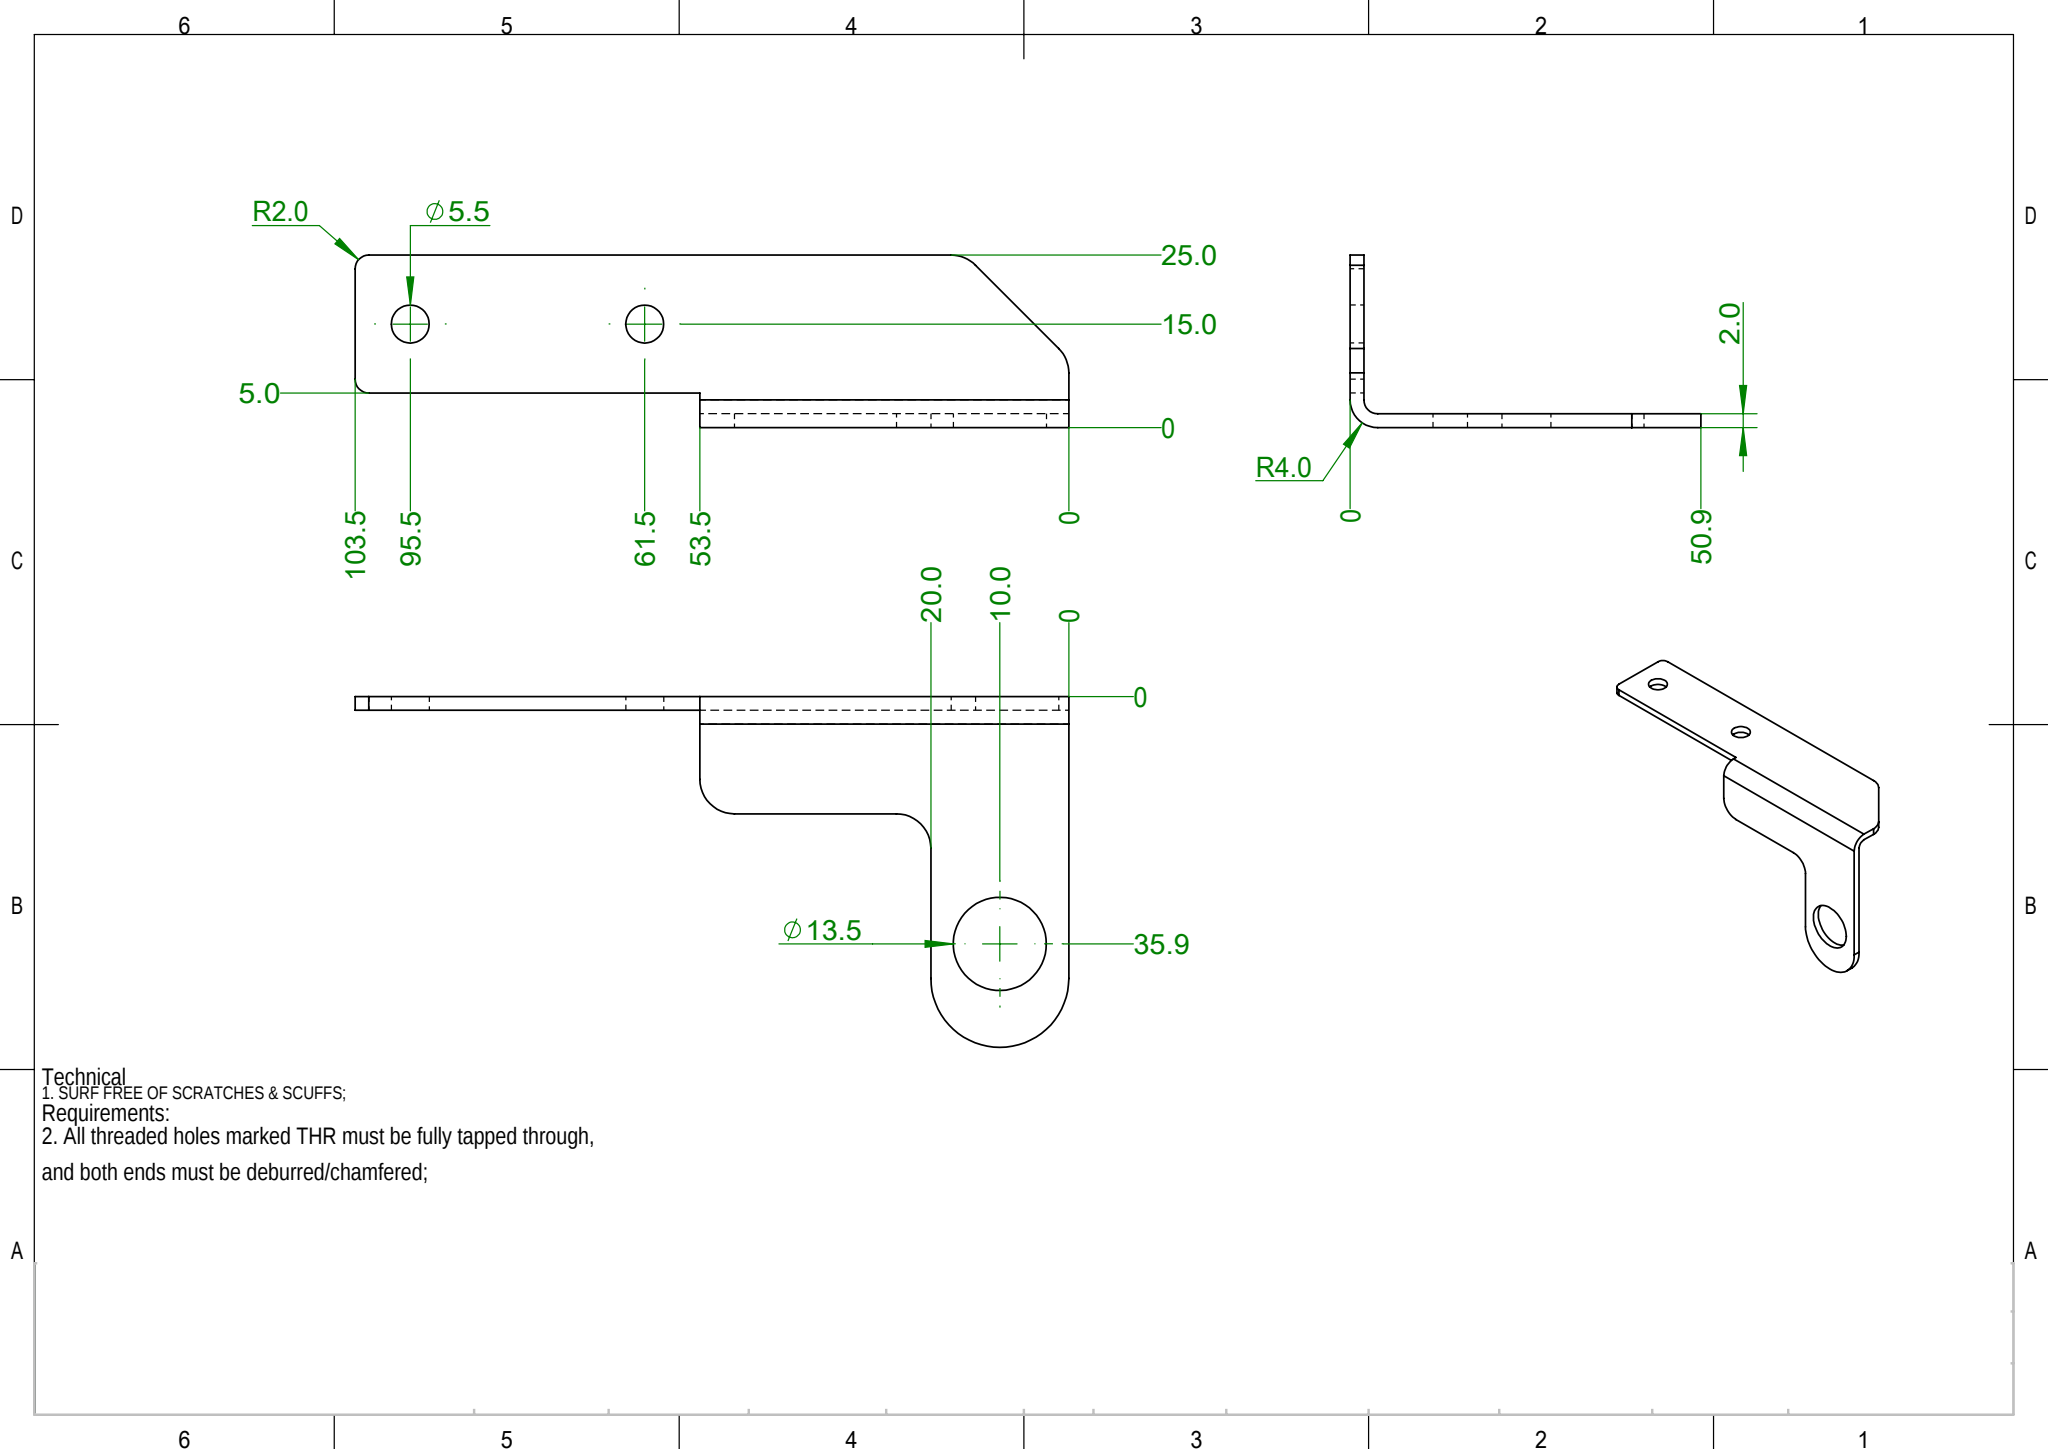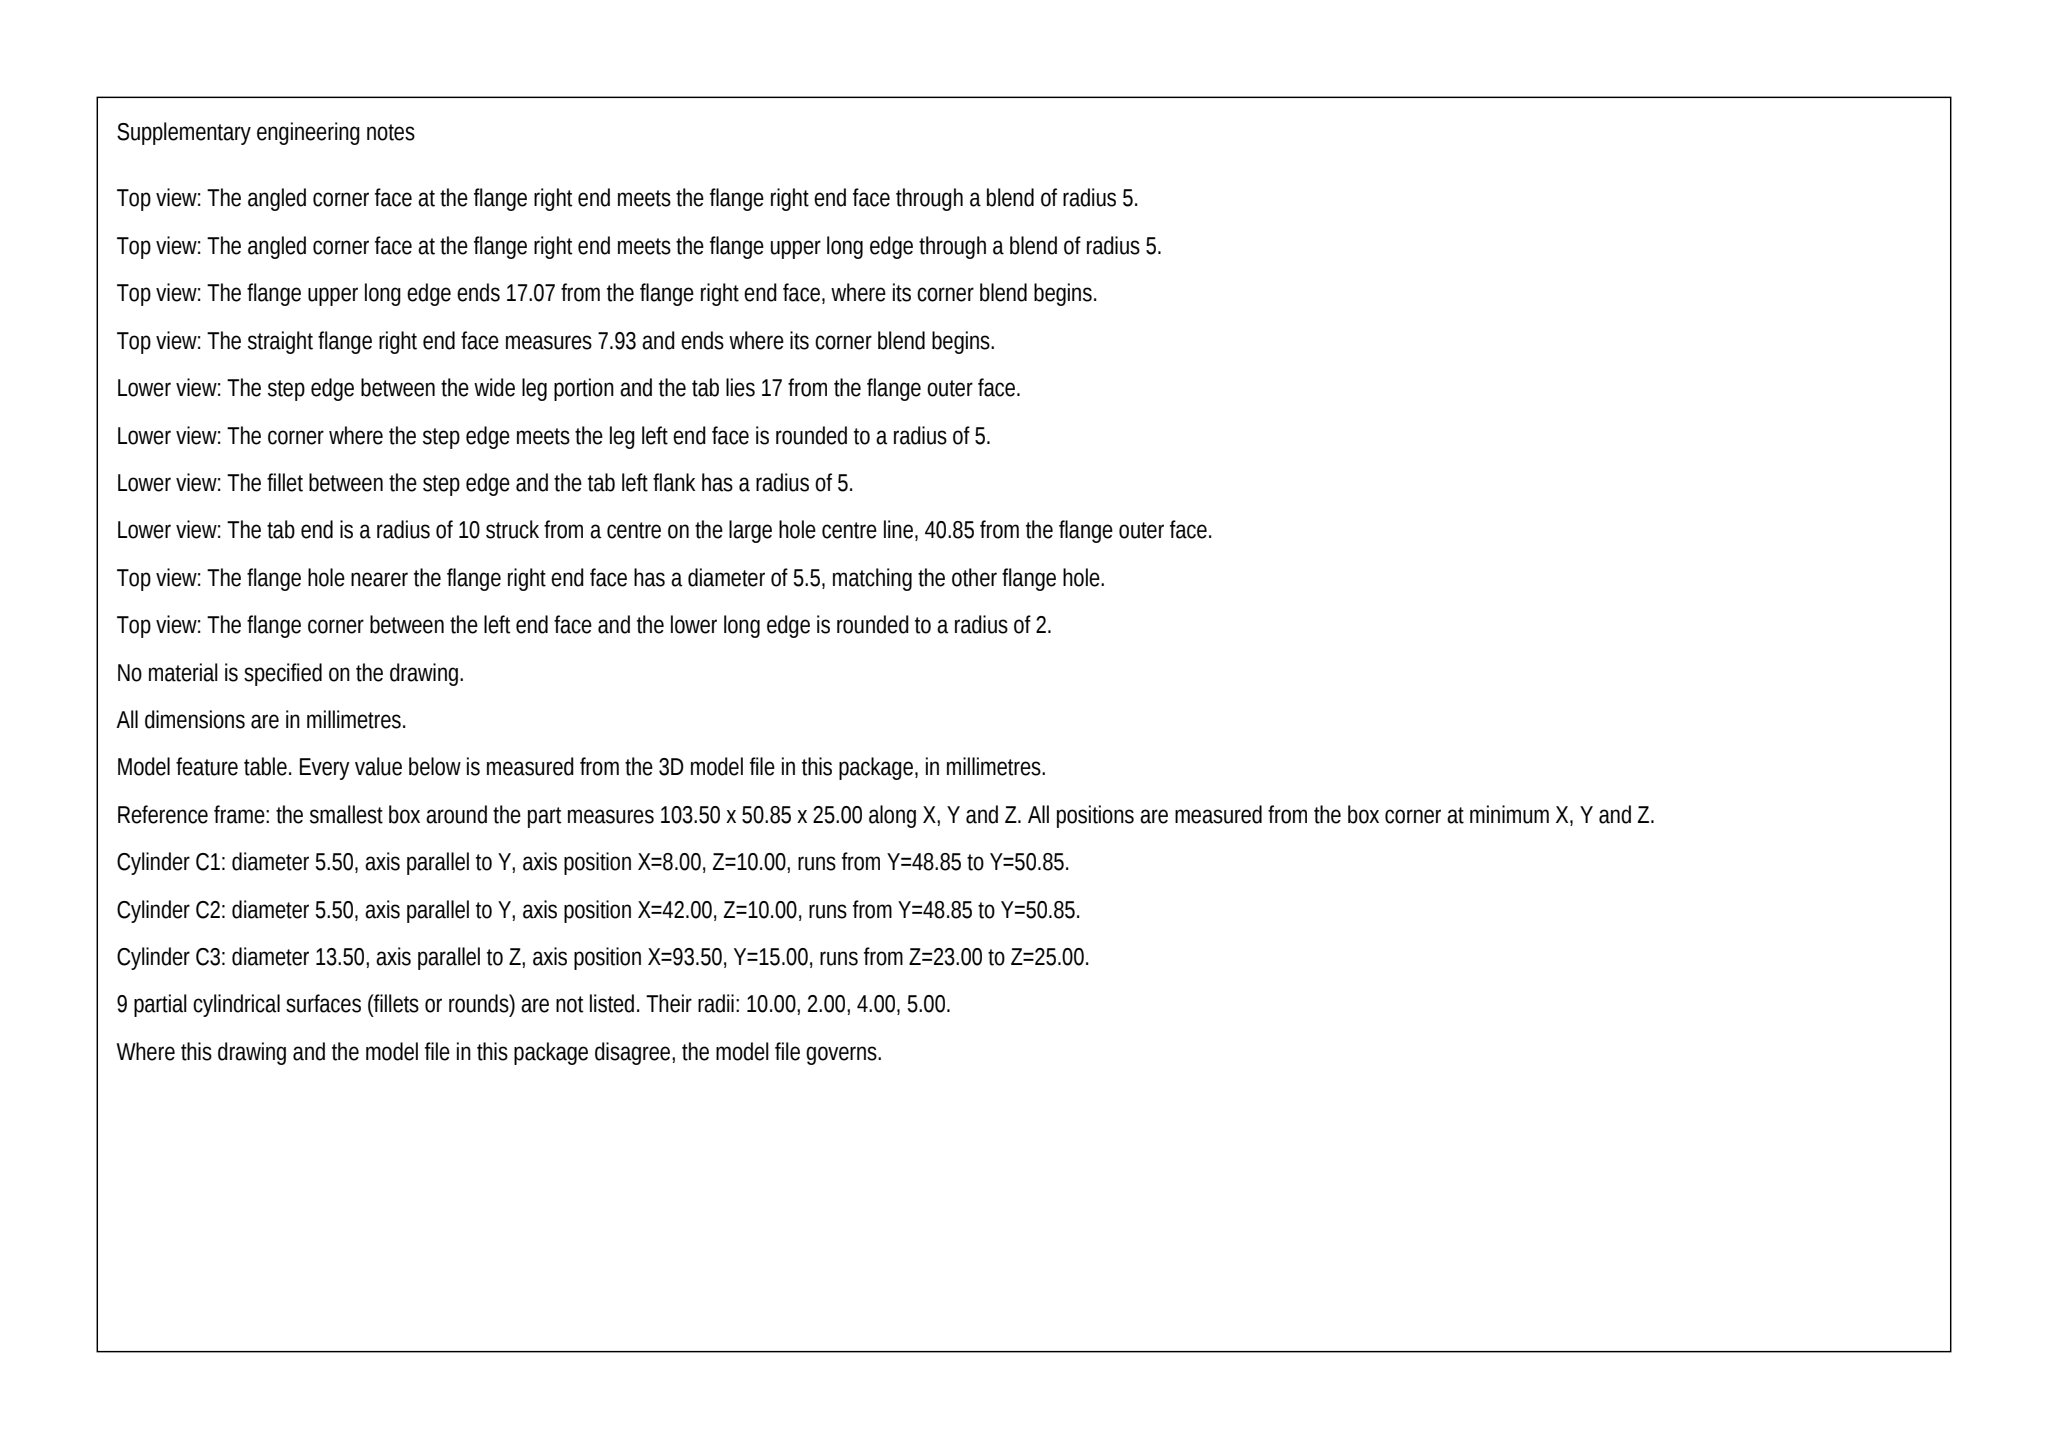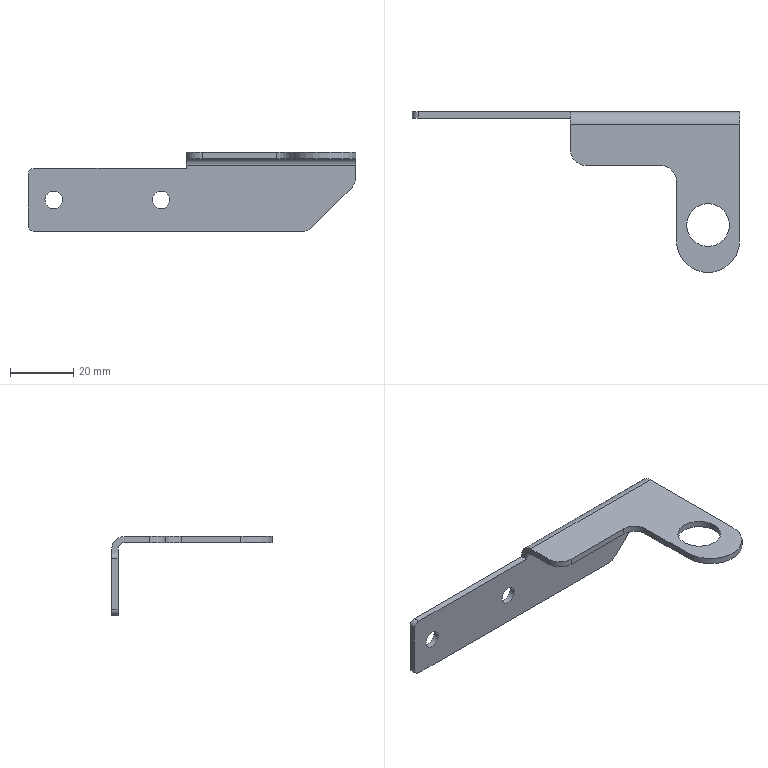Part | SolidWorks | mm | 1 solid | 27 faces | box 103.5 x 50.85 x 25 mm | volume 6798 mm3 | cylinder 15 | plane 12 | commonest cylinder face diameters 5.5 x4 10 x4 4 x3 13.5 x2 20 x1 8 x1
Drawing notes:
FRONT VIEW: 45° CORNER, SHARP PTS AT X-ORD 15.0 & Z-ORD 10.0 | from the solid: R5 fillet centers (86.43,z5.0) & (98.5,z17.07) -> ord (17.07,20)&(5.0,7.93); tangent line z=x+10 meets top ord 25 at x-ord 15.0 and end ord 0 at z-ord 10.0 (45°)
R5.0 TANGENT FILLETS BOTH ENDS OF 45° FLANGE EDGE, FRONT VIEW | from the solid: cylinders dia 10.0 axis y at (86.43,z=5.0) and (98.5,z=17.07), len 2.0 = plate thk
TOP VIEW: R5.0 OUTSIDE CNR AT PLATE FRONT, R5.0 FILLET AT TAB ROOT | from the solid: cylinders dia 10.0 axis z at (55,38.85) -> ord (48.5,12.0) tangent to x-ord 53.5 & y-ord 17.0; at (78.5,28.85) -> ord (25.0,22.0) tangent to x-ord 20.0 & y-ord 17.0
TOP VIEW: PLATE FRONT EDGE 17.0 FROM 0 ORD (PLATE DEPTH 17.0) | from the solid: plane y=33.85 vs datum face y=50.85 (y-ord 0, hole ord 35.9 = 50.85-15.0) -> 17.0
TOP VIEW TAB END: FULL RND R10, CTR X-ORD 10.0, 40.9 FROM 0 Y-ORD | from the solid: cyl dia 20.0 axis z at (93.5,10.0) -> R10; x-datum 103.5-93.5=10.0; y-datum 50.85-10.0=40.85
2X Ø5.5 THRU (X-ORD 95.5 & 61.5) | from the solid: two cyls dia 5.5 axis y at x=8.0 and x=42.0, len 2.0 (full thk)
2X R2.0 CORNER FILLETS AT BOTH ENDS OF VERTICAL PLATE LEFT-HAND EDGE (X-ORD 103.5); FILLET CENTRES 2.0 IN FROM THAT EDGE, 2.0 FROM EACH ADJACENT PLATE EDGE | from the solid: cylinders dia 4.0 axis y at [2.0, -, 2.0] and [2.0, -, 18.0], length 2.0 (plate thickness) - two R2.0 fillets on the left edge